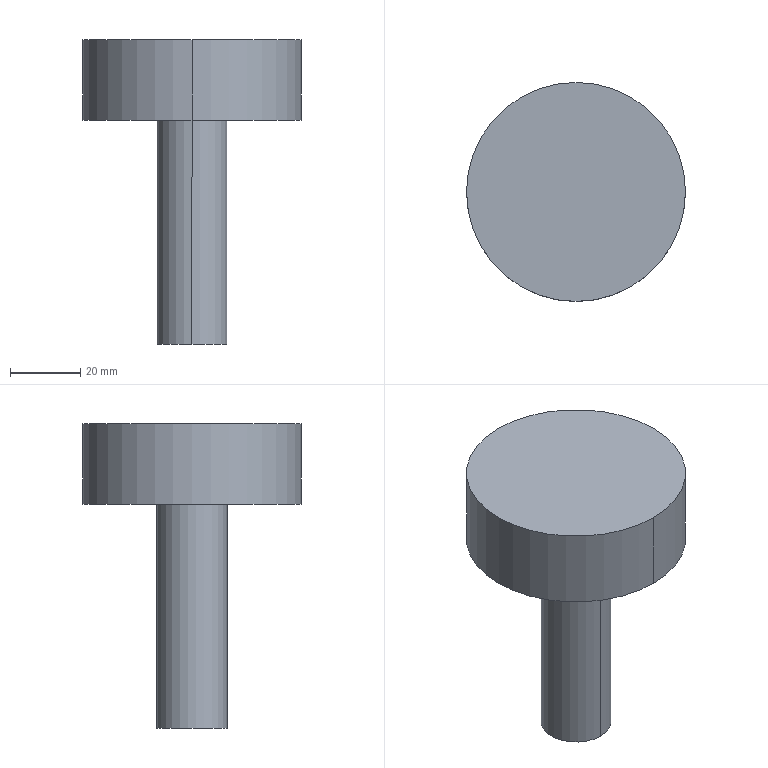Component | SolidWorks | NewCurveBenderSDAT63x45x45Cylinder-DoubleWheel-1_NewCurveBenderSDATS-63x45x45-B4545_r_3-DoubleWheel-1 | 1 solid | 7 faces | box 62.5 x 62.5 x 87 mm | volume 90669 mm3 | cylinder 4 | plane 3 | commonest cylinder face diameters 62.5 x2 20 x2
build123d program:
from build123d import *


with BuildPart() as part:
    # Sketch1 → Revolve1 (revolve)
    with BuildSketch(Plane.XY, mode=Mode.PRIVATE) as revolve1_sk:
        Polygon((122, 0), (122, 10), (186, 10), (186, 31.25), (209, 31.25), (209, 0), align=None)
    revolve(revolve1_sk.sketch.rotate(Axis((209, 0, 0), (-1, 0, 0)), 270), axis=Axis((209, 0, 0), (-1, 0, 0)))


solid = part.part

# Placed as in the assembly
solid = solid.moved(Location((0, 47, 237.459), (0, -90, 0)))
STEP:
#1=COLOUR_RGB('',0.7922,0.8196,0.9333);
#2=FILL_AREA_STYLE_COLOUR('',#1);
#3=FILL_AREA_STYLE('',(#2));
#4=SURFACE_STYLE_FILL_AREA(#3);
#5=SURFACE_SIDE_STYLE('',(#4));
#6=SURFACE_STYLE_USAGE(.BOTH.,#5);
#7=PRESENTATION_STYLE_ASSIGNMENT((#6));
#8=CARTESIAN_POINT('',(-0.,0.6201,17.577));
#9=VERTEX_POINT('',#8);
#10=CARTESIAN_POINT('',(-0.,3.081,17.577));
#11=VERTEX_POINT('',#10);
#12=CARTESIAN_POINT('',(-0.,1.85,17.577));
#13=DIRECTION('',(-0.,0.,-1.));
#14=DIRECTION('',(0.,-1.,0.));
#15=AXIS2_PLACEMENT_3D('',#12,#13,#14);
#16=CIRCLE('',#15,1.23);
#17=EDGE_CURVE('',#9,#11,#16,.T.);
#18=ORIENTED_EDGE('',*,*,#17,.T.);
#19=CARTESIAN_POINT('',(-0.,3.081,16.672));
#20=VERTEX_POINT('',#19);
#21=CARTESIAN_POINT('',(-0.,3.081,17.577));
#22=DIRECTION('',(-0.,0.,-1.));
#23=VECTOR('',#22,39.37);
#24=LINE('',#21,#23);
#25=EDGE_CURVE('',#11,#20,#24,.T.);
#26=ORIENTED_EDGE('',*,*,#25,.T.);
#27=CARTESIAN_POINT('',(-0.,0.6201,16.672));
#28=VERTEX_POINT('',#27);
#29=CARTESIAN_POINT('',(-0.,1.85,16.672));
#30=DIRECTION('',(-0.,0.,-1.));
#31=DIRECTION('',(0.,-1.,0.));
#32=AXIS2_PLACEMENT_3D('',#29,#30,#31);
#33=CIRCLE('',#32,1.23);
#34=EDGE_CURVE('',#28,#20,#33,.T.);
#35=ORIENTED_EDGE('',*,*,#34,.F.);
#36=CARTESIAN_POINT('',(-0.,0.6201,17.577));
#37=DIRECTION('',(-0.,0.,-1.));
#38=VECTOR('',#37,39.37);
#39=LINE('',#36,#38);
#40=EDGE_CURVE('',#9,#28,#39,.T.);
#41=ORIENTED_EDGE('',*,*,#40,.F.);
#42=EDGE_LOOP('',(#18,#26,#35,#41));
#43=FACE_OUTER_BOUND('',#42,.T.);
#44=CARTESIAN_POINT('',(-0.,1.85,17.577));
#45=DIRECTION('',(-0.,0.,-1.));
#46=DIRECTION('',(0.,-1.,0.));
#47=AXIS2_PLACEMENT_3D('',#44,#45,#46);
#48=CYLINDRICAL_SURFACE('',#47,1.23);
#49=ADVANCED_FACE('',(#43),#48,.T.);
#50=CARTESIAN_POINT('',(-0.,1.457,16.672));
#51=VERTEX_POINT('',#50);
#52=CARTESIAN_POINT('',(-0.,2.244,16.672));
#53=VERTEX_POINT('',#52);
#54=CARTESIAN_POINT('',(-0.,1.85,16.672));
#55=DIRECTION('',(-0.,0.,-1.));
#56=DIRECTION('',(0.,-1.,0.));
#57=AXIS2_PLACEMENT_3D('',#54,#55,#56);
#58=CIRCLE('',#57,0.3937);
#59=EDGE_CURVE('',#51,#53,#58,.T.);
#60=ORIENTED_EDGE('',*,*,#59,.T.);
#61=CARTESIAN_POINT('',(-0.,2.244,14.152));
#62=VERTEX_POINT('',#61);
#63=CARTESIAN_POINT('',(-0.,2.244,17.577));
#64=DIRECTION('',(-0.,0.,-1.));
#65=VECTOR('',#64,39.37);
#66=LINE('',#63,#65);
#67=EDGE_CURVE('',#53,#62,#66,.T.);
#68=ORIENTED_EDGE('',*,*,#67,.T.);
#69=CARTESIAN_POINT('',(-0.,1.457,14.152));
#70=VERTEX_POINT('',#69);
#71=CARTESIAN_POINT('',(-0.,1.85,14.152));
#72=DIRECTION('',(-0.,0.,-1.));
#73=DIRECTION('',(0.,-1.,0.));
#74=AXIS2_PLACEMENT_3D('',#71,#72,#73);
#75=CIRCLE('',#74,0.3937);
#76=EDGE_CURVE('',#70,#62,#75,.T.);
#77=ORIENTED_EDGE('',*,*,#76,.F.);
#78=CARTESIAN_POINT('',(-0.,1.457,17.577));
#79=DIRECTION('',(-0.,0.,-1.));
#80=VECTOR('',#79,39.37);
#81=LINE('',#78,#80);
#82=EDGE_CURVE('',#51,#70,#81,.T.);
#83=ORIENTED_EDGE('',*,*,#82,.F.);
#84=EDGE_LOOP('',(#60,#68,#77,#83));
#85=FACE_OUTER_BOUND('',#84,.T.);
#86=CARTESIAN_POINT('',(-0.,1.85,17.577));
#87=DIRECTION('',(-0.,0.,-1.));
#88=DIRECTION('',(0.,-1.,0.));
#89=AXIS2_PLACEMENT_3D('',#86,#87,#88);
#90=CYLINDRICAL_SURFACE('',#89,0.3937);
#91=ADVANCED_FACE('',(#85),#90,.T.);
#92=ORIENTED_EDGE('',*,*,#76,.T.);
#93=CARTESIAN_POINT('',(-0.,1.85,14.152));
#94=DIRECTION('',(-0.,0.,-1.));
#95=DIRECTION('',(0.,-1.,0.));
#96=AXIS2_PLACEMENT_3D('',#93,#94,#95);
#97=CIRCLE('',#96,0.3937);
#98=EDGE_CURVE('',#62,#70,#97,.T.);
#99=ORIENTED_EDGE('',*,*,#98,.T.);
#100=EDGE_LOOP('',(#92,#99));
#101=FACE_OUTER_BOUND('',#100,.T.);
#102=CARTESIAN_POINT('',(-0.,1.85,14.152));
#103=DIRECTION('',(0.,-0.,1.));
#104=DIRECTION('',(-0.,1.,0.));
#105=AXIS2_PLACEMENT_3D('',#102,#103,#104);
#106=PLANE('',#105);
#107=ADVANCED_FACE('',(#101),#106,.F.);
#108=ORIENTED_EDGE('',*,*,#67,.F.);
#109=CARTESIAN_POINT('',(-0.,1.85,16.672));
#110=DIRECTION('',(-0.,0.,-1.));
#111=DIRECTION('',(0.,-1.,0.));
#112=AXIS2_PLACEMENT_3D('',#109,#110,#111);
#113=CIRCLE('',#112,0.3937);
#114=EDGE_CURVE('',#53,#51,#113,.T.);
#115=ORIENTED_EDGE('',*,*,#114,.T.);
#116=ORIENTED_EDGE('',*,*,#82,.T.);
#117=ORIENTED_EDGE('',*,*,#98,.F.);
#118=EDGE_LOOP('',(#108,#115,#116,#117));
#119=FACE_OUTER_BOUND('',#118,.T.);
#120=CARTESIAN_POINT('',(-0.,1.85,17.577));
#121=DIRECTION('',(-0.,0.,-1.));
#122=DIRECTION('',(0.,-1.,0.));
#123=AXIS2_PLACEMENT_3D('',#120,#121,#122);
#124=CYLINDRICAL_SURFACE('',#123,0.3937);
#125=ADVANCED_FACE('',(#119),#124,.T.);
#126=ORIENTED_EDGE('',*,*,#59,.F.);
#127=ORIENTED_EDGE('',*,*,#114,.F.);
#128=EDGE_LOOP('',(#126,#127));
#129=FACE_BOUND('',#128,.T.);
#130=ORIENTED_EDGE('',*,*,#34,.T.);
#131=CARTESIAN_POINT('',(-0.,1.85,16.672));
#132=DIRECTION('',(-0.,0.,-1.));
#133=DIRECTION('',(0.,-1.,0.));
#134=AXIS2_PLACEMENT_3D('',#131,#132,#133);
#135=CIRCLE('',#134,1.23);
#136=EDGE_CURVE('',#20,#28,#135,.T.);
#137=ORIENTED_EDGE('',*,*,#136,.T.);
#138=EDGE_LOOP('',(#130,#137));
#139=FACE_OUTER_BOUND('',#138,.T.);
#140=CARTESIAN_POINT('',(-0.3937,1.85,16.672));
#141=DIRECTION('',(0.,-0.,1.));
#142=DIRECTION('',(-0.,1.,0.));
#143=AXIS2_PLACEMENT_3D('',#140,#141,#142);
#144=PLANE('',#143);
#145=ADVANCED_FACE('',(#129,#139),#144,.F.);
#146=ORIENTED_EDGE('',*,*,#25,.F.);
#147=CARTESIAN_POINT('',(-0.,1.85,17.577));
#148=DIRECTION('',(-0.,0.,-1.));
#149=DIRECTION('',(0.,-1.,0.));
#150=AXIS2_PLACEMENT_3D('',#147,#148,#149);
#151=CIRCLE('',#150,1.23);
#152=EDGE_CURVE('',#11,#9,#151,.T.);
#153=ORIENTED_EDGE('',*,*,#152,.T.);
#154=ORIENTED_EDGE('',*,*,#40,.T.);
#155=ORIENTED_EDGE('',*,*,#136,.F.);
#156=EDGE_LOOP('',(#146,#153,#154,#155));
#157=FACE_OUTER_BOUND('',#156,.T.);
#158=CARTESIAN_POINT('',(-0.,1.85,17.577));
#159=DIRECTION('',(-0.,0.,-1.));
#160=DIRECTION('',(0.,-1.,0.));
#161=AXIS2_PLACEMENT_3D('',#158,#159,#160);
#162=CYLINDRICAL_SURFACE('',#161,1.23);
#163=ADVANCED_FACE('',(#157),#162,.T.);
#164=ORIENTED_EDGE('',*,*,#17,.F.);
#165=ORIENTED_EDGE('',*,*,#152,.F.);
#166=EDGE_LOOP('',(#164,#165));
#167=FACE_OUTER_BOUND('',#166,.T.);
#168=CARTESIAN_POINT('',(-1.23,1.85,17.577));
#169=DIRECTION('',(-0.,0.,-1.));
#170=DIRECTION('',(0.,-1.,-0.));
#171=AXIS2_PLACEMENT_3D('',#168,#169,#170);
#172=PLANE('',#171);
#173=ADVANCED_FACE('',(#167),#172,.F.);
#174=CLOSED_SHELL('',(#49,#91,#107,#125,#145,#163,#173));
#175=MANIFOLD_SOLID_BREP('',#174);
#176=STYLED_ITEM('',(#7),#175);
#177=PRESENTATION_LAYER_ASSIGNMENT('','',(#176));
#178=CARTESIAN_POINT('',(0.,0.,0.));
#179=DIRECTION('',(0.,0.,1.));
#180=DIRECTION('',(1.,0.,0.));
#181=AXIS2_PLACEMENT_3D('',#178,#179,#180);
#182=(LENGTH_UNIT()NAMED_UNIT(*)SI_UNIT($,.METRE.));
#183=LENGTH_MEASURE_WITH_UNIT(LENGTH_MEASURE(0.0254),#182);
#184=DIMENSIONAL_EXPONENTS(1.,0.,0.,0.,0.,0.,0.);
#185=(CONVERSION_BASED_UNIT('',#183)LENGTH_UNIT()NAMED_UNIT(#184));
#186=UNCERTAINTY_MEASURE_WITH_UNIT(LENGTH_MEASURE(0.00001),#185,'','');
#187=(NAMED_UNIT(*)PLANE_ANGLE_UNIT()SI_UNIT($,.RADIAN.));
#188=(NAMED_UNIT(*)SI_UNIT($,.STERADIAN.)SOLID_ANGLE_UNIT());
#189=(GEOMETRIC_REPRESENTATION_CONTEXT(3)GLOBAL_UNCERTAINTY_ASSIGNED_CONTEXT((#186))GLOBAL_UNIT_ASSIGNED_CONTEXT((#185,#187,#188))REPRESENTATION_CONTEXT('',''));
#190=ADVANCED_BREP_SHAPE_REPRESENTATION('',(#175,#181),#189);
#191=(LENGTH_UNIT()NAMED_UNIT(*)SI_UNIT($,.METRE.));
#192=LENGTH_MEASURE_WITH_UNIT(LENGTH_MEASURE(0.0254),#191);
#193=DIMENSIONAL_EXPONENTS(1.,0.,0.,0.,0.,0.,0.);
#194=(CONVERSION_BASED_UNIT('',#192)LENGTH_UNIT()NAMED_UNIT(#193));
#195=UNCERTAINTY_MEASURE_WITH_UNIT(LENGTH_MEASURE(0.00001),#194,'','');
#196=(NAMED_UNIT(*)PLANE_ANGLE_UNIT()SI_UNIT($,.RADIAN.));
#197=(NAMED_UNIT(*)SI_UNIT($,.STERADIAN.)SOLID_ANGLE_UNIT());
#198=(GEOMETRIC_REPRESENTATION_CONTEXT(3)GLOBAL_UNCERTAINTY_ASSIGNED_CONTEXT((#195))GLOBAL_UNIT_ASSIGNED_CONTEXT((#194,#196,#197))REPRESENTATION_CONTEXT('',''));
#199=MECHANICAL_DESIGN_GEOMETRIC_PRESENTATION_REPRESENTATION('',(#176),#198);